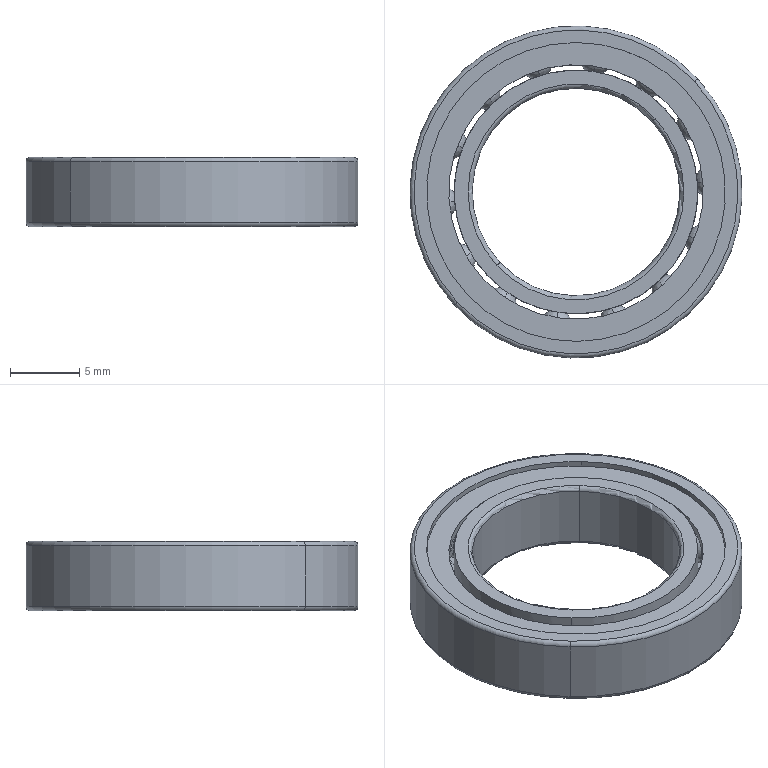Component | SolidWorks | 04DeepGrooveBallBearing61802-2Z-4 | 1 solid | 225 faces | volume 963 mm3 | sphere 112 | torus 53 | plane 36 | cylinder 24 | commonest cylinder face diameters 21.6 x8 18.386 x4 17.6 x4 15 x2 24 x2 20.255 x2 18.945 x2